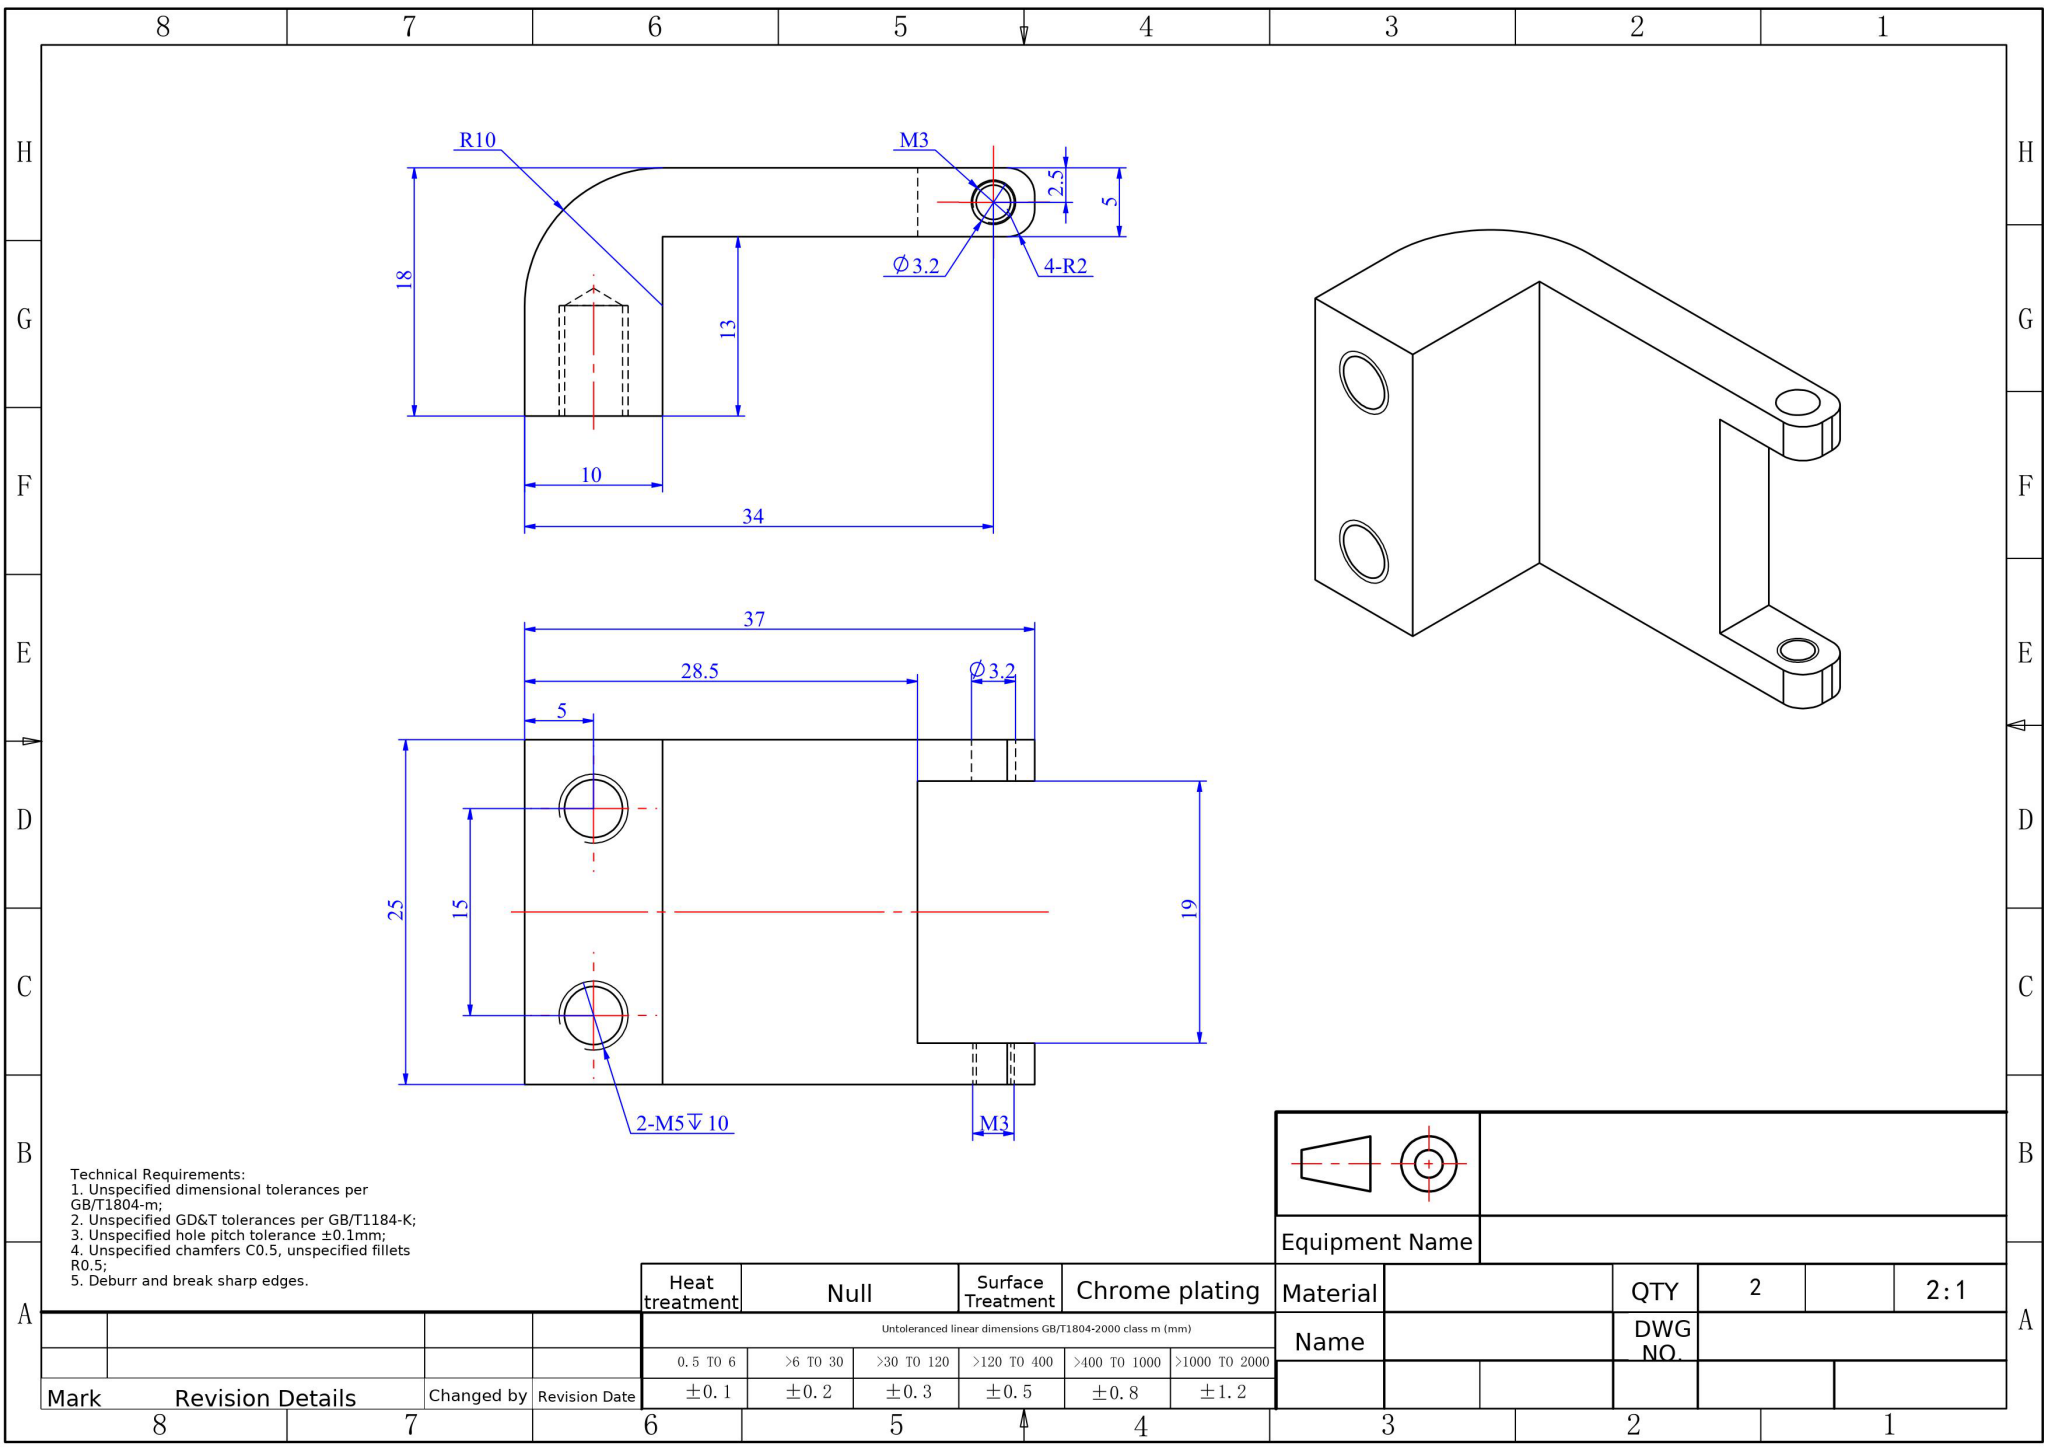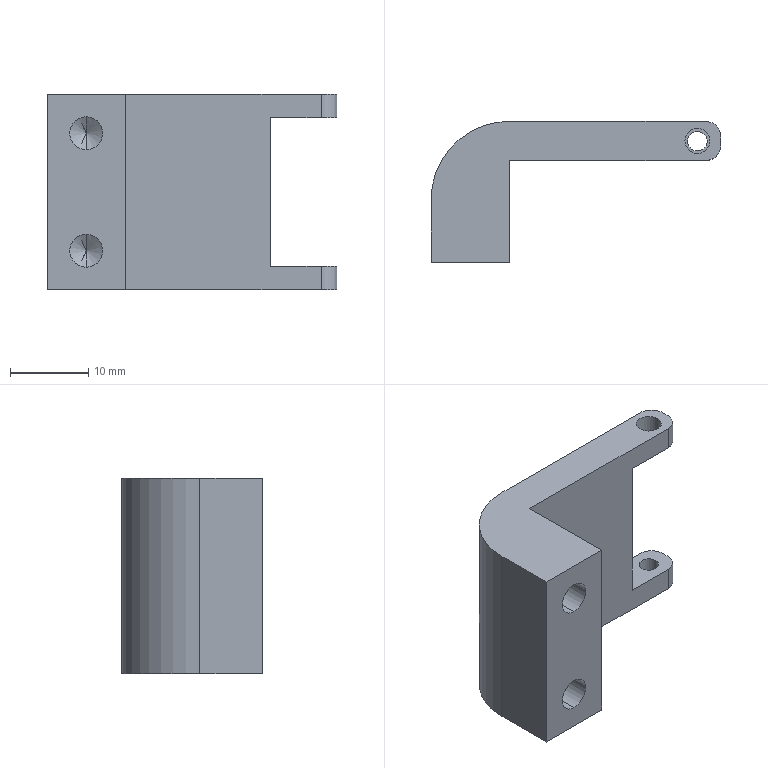Part | NX | mm | 1 solid | 29 faces | box 37 x 18 x 25 mm | volume 6249 mm3 | cylinder 13 | plane 12 | cone 4 | commonest cylinder face diameters 4.2 x4 4 x4 2.5 x2 3.2 x2 20 x1
STEP:
#1=COLOUR_RGB('',0.7922,0.8196,0.9333);
#2=FILL_AREA_STYLE_COLOUR('',#1);
#3=FILL_AREA_STYLE('',(#2));
#4=SURFACE_STYLE_FILL_AREA(#3);
#5=SURFACE_SIDE_STYLE('',(#4));
#6=SURFACE_STYLE_USAGE(.BOTH.,#5);
#7=PRESENTATION_STYLE_ASSIGNMENT((#6));
#8=CARTESIAN_POINT('',(32.75,15.498,-12.5));
#9=VERTEX_POINT('',#8);
#10=CARTESIAN_POINT('',(35.25,15.498,-12.5));
#11=VERTEX_POINT('',#10);
#12=CARTESIAN_POINT('',(34.,15.498,-12.5));
#13=DIRECTION('',(0.,0.,1.));
#14=DIRECTION('',(1.,0.,0.));
#15=AXIS2_PLACEMENT_3D('',#12,#13,#14);
#16=CIRCLE('',#15,1.25);
#17=EDGE_CURVE('',#9,#11,#16,.T.);
#18=ORIENTED_EDGE('',*,*,#17,.F.);
#19=CARTESIAN_POINT('',(32.75,15.498,-9.5));
#20=VERTEX_POINT('',#19);
#21=CARTESIAN_POINT('',(32.75,15.498,-9.5));
#22=DIRECTION('',(0.,0.,1.));
#23=VECTOR('',#22,1000.);
#24=LINE('',#21,#23);
#25=EDGE_CURVE('',#9,#20,#24,.T.);
#26=ORIENTED_EDGE('',*,*,#25,.T.);
#27=CARTESIAN_POINT('',(35.25,15.498,-9.5));
#28=VERTEX_POINT('',#27);
#29=CARTESIAN_POINT('',(34.,15.498,-9.5));
#30=DIRECTION('',(0.,0.,1.));
#31=DIRECTION('',(1.,0.,0.));
#32=AXIS2_PLACEMENT_3D('',#29,#30,#31);
#33=CIRCLE('',#32,1.25);
#34=EDGE_CURVE('',#20,#28,#33,.T.);
#35=ORIENTED_EDGE('',*,*,#34,.T.);
#36=CARTESIAN_POINT('',(35.25,15.498,-9.5));
#37=DIRECTION('',(0.,0.,1.));
#38=VECTOR('',#37,1000.);
#39=LINE('',#36,#38);
#40=EDGE_CURVE('',#11,#28,#39,.T.);
#41=ORIENTED_EDGE('',*,*,#40,.F.);
#42=EDGE_LOOP('',(#18,#26,#35,#41));
#43=FACE_OUTER_BOUND('',#42,.T.);
#44=CARTESIAN_POINT('',(34.,15.498,-9.5));
#45=DIRECTION('',(0.,0.,1.));
#46=DIRECTION('',(1.,0.,0.));
#47=AXIS2_PLACEMENT_3D('',#44,#45,#46);
#48=CYLINDRICAL_SURFACE('',#47,1.25);
#49=ADVANCED_FACE('',(#43),#48,.F.);
#50=CARTESIAN_POINT('',(5.,8.,9.6));
#51=VERTEX_POINT('',#50);
#52=CARTESIAN_POINT('',(5.,8.,5.4));
#53=VERTEX_POINT('',#52);
#54=CARTESIAN_POINT('',(5.,8.,7.5));
#55=DIRECTION('',(0.,-1.,0.));
#56=DIRECTION('',(0.,0.,-1.));
#57=AXIS2_PLACEMENT_3D('',#54,#55,#56);
#58=CIRCLE('',#57,2.1);
#59=EDGE_CURVE('',#51,#53,#58,.T.);
#60=ORIENTED_EDGE('',*,*,#59,.F.);
#61=CARTESIAN_POINT('',(5.,0.,9.6));
#62=VERTEX_POINT('',#61);
#63=CARTESIAN_POINT('',(5.,0.,9.6));
#64=DIRECTION('',(0.,-1.,0.));
#65=VECTOR('',#64,1000.);
#66=LINE('',#63,#65);
#67=EDGE_CURVE('',#51,#62,#66,.T.);
#68=ORIENTED_EDGE('',*,*,#67,.T.);
#69=CARTESIAN_POINT('',(5.,0.,5.4));
#70=VERTEX_POINT('',#69);
#71=CARTESIAN_POINT('',(5.,0.,7.5));
#72=DIRECTION('',(0.,-1.,0.));
#73=DIRECTION('',(0.,0.,-1.));
#74=AXIS2_PLACEMENT_3D('',#71,#72,#73);
#75=CIRCLE('',#74,2.1);
#76=EDGE_CURVE('',#62,#70,#75,.T.);
#77=ORIENTED_EDGE('',*,*,#76,.T.);
#78=CARTESIAN_POINT('',(5.,0.,5.4));
#79=DIRECTION('',(0.,-1.,0.));
#80=VECTOR('',#79,1000.);
#81=LINE('',#78,#80);
#82=EDGE_CURVE('',#53,#70,#81,.T.);
#83=ORIENTED_EDGE('',*,*,#82,.F.);
#84=EDGE_LOOP('',(#60,#68,#77,#83));
#85=FACE_OUTER_BOUND('',#84,.T.);
#86=CARTESIAN_POINT('',(5.,0.,7.5));
#87=DIRECTION('',(0.,-1.,0.));
#88=DIRECTION('',(0.,0.,-1.));
#89=AXIS2_PLACEMENT_3D('',#86,#87,#88);
#90=CYLINDRICAL_SURFACE('',#89,2.1);
#91=ADVANCED_FACE('',(#85),#90,.F.);
#92=CARTESIAN_POINT('',(5.,9.262,7.5));
#93=VERTEX_POINT('',#92);
#94=CARTESIAN_POINT('',(5.,8.,5.4));
#95=DIRECTION('',(0.,-0.515,-0.8572));
#96=VECTOR('',#95,1000.);
#97=LINE('',#94,#96);
#98=EDGE_CURVE('',#93,#53,#97,.T.);
#99=ORIENTED_EDGE('',*,*,#98,.F.);
#100=CARTESIAN_POINT('',(5.,8.,9.6));
#101=DIRECTION('',(0.,-0.515,0.8572));
#102=VECTOR('',#101,1000.);
#103=LINE('',#100,#102);
#104=EDGE_CURVE('',#93,#51,#103,.T.);
#105=ORIENTED_EDGE('',*,*,#104,.T.);
#106=ORIENTED_EDGE('',*,*,#59,.T.);
#107=EDGE_LOOP('',(#99,#105,#106));
#108=FACE_OUTER_BOUND('',#107,.T.);
#109=CARTESIAN_POINT('',(5.,8.,7.5));
#110=DIRECTION('',(0.,-1.,0.));
#111=DIRECTION('',(0.,0.,-1.));
#112=AXIS2_PLACEMENT_3D('',#109,#110,#111);
#113=CONICAL_SURFACE('',#112,2.1,1.03);
#114=ADVANCED_FACE('',(#108),#113,.F.);
#115=CARTESIAN_POINT('',(5.,8.,-5.4));
#116=VERTEX_POINT('',#115);
#117=CARTESIAN_POINT('',(5.,8.,-9.6));
#118=VERTEX_POINT('',#117);
#119=CARTESIAN_POINT('',(5.,8.,-7.5));
#120=DIRECTION('',(0.,-1.,0.));
#121=DIRECTION('',(0.,0.,-1.));
#122=AXIS2_PLACEMENT_3D('',#119,#120,#121);
#123=CIRCLE('',#122,2.1);
#124=EDGE_CURVE('',#116,#118,#123,.T.);
#125=ORIENTED_EDGE('',*,*,#124,.F.);
#126=CARTESIAN_POINT('',(5.,0.,-5.4));
#127=VERTEX_POINT('',#126);
#128=CARTESIAN_POINT('',(5.,0.,-5.4));
#129=DIRECTION('',(0.,-1.,0.));
#130=VECTOR('',#129,1000.);
#131=LINE('',#128,#130);
#132=EDGE_CURVE('',#116,#127,#131,.T.);
#133=ORIENTED_EDGE('',*,*,#132,.T.);
#134=CARTESIAN_POINT('',(5.,0.,-9.6));
#135=VERTEX_POINT('',#134);
#136=CARTESIAN_POINT('',(5.,0.,-7.5));
#137=DIRECTION('',(0.,-1.,0.));
#138=DIRECTION('',(0.,0.,-1.));
#139=AXIS2_PLACEMENT_3D('',#136,#137,#138);
#140=CIRCLE('',#139,2.1);
#141=EDGE_CURVE('',#127,#135,#140,.T.);
#142=ORIENTED_EDGE('',*,*,#141,.T.);
#143=CARTESIAN_POINT('',(5.,0.,-9.6));
#144=DIRECTION('',(0.,-1.,0.));
#145=VECTOR('',#144,1000.);
#146=LINE('',#143,#145);
#147=EDGE_CURVE('',#118,#135,#146,.T.);
#148=ORIENTED_EDGE('',*,*,#147,.F.);
#149=EDGE_LOOP('',(#125,#133,#142,#148));
#150=FACE_OUTER_BOUND('',#149,.T.);
#151=CARTESIAN_POINT('',(5.,0.,-7.5));
#152=DIRECTION('',(0.,-1.,0.));
#153=DIRECTION('',(0.,0.,-1.));
#154=AXIS2_PLACEMENT_3D('',#151,#152,#153);
#155=CYLINDRICAL_SURFACE('',#154,2.1);
#156=ADVANCED_FACE('',(#150),#155,.F.);
#157=CARTESIAN_POINT('',(5.,9.262,-7.5));
#158=VERTEX_POINT('',#157);
#159=CARTESIAN_POINT('',(5.,8.,-9.6));
#160=DIRECTION('',(0.,-0.515,-0.8572));
#161=VECTOR('',#160,1000.);
#162=LINE('',#159,#161);
#163=EDGE_CURVE('',#158,#118,#162,.T.);
#164=ORIENTED_EDGE('',*,*,#163,.F.);
#165=CARTESIAN_POINT('',(5.,8.,-5.4));
#166=DIRECTION('',(0.,-0.515,0.8572));
#167=VECTOR('',#166,1000.);
#168=LINE('',#165,#167);
#169=EDGE_CURVE('',#158,#116,#168,.T.);
#170=ORIENTED_EDGE('',*,*,#169,.T.);
#171=ORIENTED_EDGE('',*,*,#124,.T.);
#172=EDGE_LOOP('',(#164,#170,#171));
#173=FACE_OUTER_BOUND('',#172,.T.);
#174=CARTESIAN_POINT('',(5.,8.,-7.5));
#175=DIRECTION('',(0.,-1.,0.));
#176=DIRECTION('',(0.,0.,-1.));
#177=AXIS2_PLACEMENT_3D('',#174,#175,#176);
#178=CONICAL_SURFACE('',#177,2.1,1.03);
#179=ADVANCED_FACE('',(#173),#178,.F.);
#180=CARTESIAN_POINT('',(32.4,15.498,9.5));
#181=VERTEX_POINT('',#180);
#182=CARTESIAN_POINT('',(35.6,15.498,9.5));
#183=VERTEX_POINT('',#182);
#184=CARTESIAN_POINT('',(34.,15.498,9.5));
#185=DIRECTION('',(0.,0.,1.));
#186=DIRECTION('',(1.,0.,0.));
#187=AXIS2_PLACEMENT_3D('',#184,#185,#186);
#188=CIRCLE('',#187,1.6);
#189=EDGE_CURVE('',#181,#183,#188,.T.);
#190=ORIENTED_EDGE('',*,*,#189,.F.);
#191=CARTESIAN_POINT('',(32.4,15.498,12.5));
#192=VERTEX_POINT('',#191);
#193=CARTESIAN_POINT('',(32.4,15.498,12.5));
#194=DIRECTION('',(0.,0.,1.));
#195=VECTOR('',#194,1000.);
#196=LINE('',#193,#195);
#197=EDGE_CURVE('',#181,#192,#196,.T.);
#198=ORIENTED_EDGE('',*,*,#197,.T.);
#199=CARTESIAN_POINT('',(35.6,15.498,12.5));
#200=VERTEX_POINT('',#199);
#201=CARTESIAN_POINT('',(34.,15.498,12.5));
#202=DIRECTION('',(0.,0.,1.));
#203=DIRECTION('',(1.,0.,0.));
#204=AXIS2_PLACEMENT_3D('',#201,#202,#203);
#205=CIRCLE('',#204,1.6);
#206=EDGE_CURVE('',#192,#200,#205,.T.);
#207=ORIENTED_EDGE('',*,*,#206,.T.);
#208=CARTESIAN_POINT('',(35.6,15.498,12.5));
#209=DIRECTION('',(0.,0.,1.));
#210=VECTOR('',#209,1000.);
#211=LINE('',#208,#210);
#212=EDGE_CURVE('',#183,#200,#211,.T.);
#213=ORIENTED_EDGE('',*,*,#212,.F.);
#214=EDGE_LOOP('',(#190,#198,#207,#213));
#215=FACE_OUTER_BOUND('',#214,.T.);
#216=CARTESIAN_POINT('',(34.,15.498,12.5));
#217=DIRECTION('',(0.,0.,1.));
#218=DIRECTION('',(1.,0.,0.));
#219=AXIS2_PLACEMENT_3D('',#216,#217,#218);
#220=CYLINDRICAL_SURFACE('',#219,1.6);
#221=ADVANCED_FACE('',(#215),#220,.F.);
#222=CARTESIAN_POINT('',(10.,13.,12.5));
#223=VERTEX_POINT('',#222);
#224=CARTESIAN_POINT('',(35.,13.,12.5));
#225=VERTEX_POINT('',#224);
#226=CARTESIAN_POINT('',(10.,13.,12.5));
#227=DIRECTION('',(1.,-0.,0.));
#228=VECTOR('',#227,1000.);
#229=LINE('',#226,#228);
#230=EDGE_CURVE('',#223,#225,#229,.T.);
#231=ORIENTED_EDGE('',*,*,#230,.T.);
#232=CARTESIAN_POINT('',(37.,15.,12.5));
#233=VERTEX_POINT('',#232);
#234=CARTESIAN_POINT('',(35.,15.,12.5));
#235=DIRECTION('',(0.,0.,1.));
#236=DIRECTION('',(-1.,0.,0.));
#237=AXIS2_PLACEMENT_3D('',#234,#235,#236);
#238=CIRCLE('',#237,2.);
#239=EDGE_CURVE('',#225,#233,#238,.T.);
#240=ORIENTED_EDGE('',*,*,#239,.T.);
#241=CARTESIAN_POINT('',(37.,16.,12.5));
#242=VERTEX_POINT('',#241);
#243=CARTESIAN_POINT('',(37.,13.,12.5));
#244=DIRECTION('',(0.,1.,0.));
#245=VECTOR('',#244,1000.);
#246=LINE('',#243,#245);
#247=EDGE_CURVE('',#233,#242,#246,.T.);
#248=ORIENTED_EDGE('',*,*,#247,.T.);
#249=CARTESIAN_POINT('',(35.,18.,12.5));
#250=VERTEX_POINT('',#249);
#251=CARTESIAN_POINT('',(35.,16.,12.5));
#252=DIRECTION('',(0.,0.,1.));
#253=DIRECTION('',(-1.,0.,0.));
#254=AXIS2_PLACEMENT_3D('',#251,#252,#253);
#255=CIRCLE('',#254,2.);
#256=EDGE_CURVE('',#242,#250,#255,.T.);
#257=ORIENTED_EDGE('',*,*,#256,.T.);
#258=CARTESIAN_POINT('',(10.,18.,12.5));
#259=VERTEX_POINT('',#258);
#260=CARTESIAN_POINT('',(37.,18.,12.5));
#261=DIRECTION('',(-1.,-0.,0.));
#262=VECTOR('',#261,1000.);
#263=LINE('',#260,#262);
#264=EDGE_CURVE('',#250,#259,#263,.T.);
#265=ORIENTED_EDGE('',*,*,#264,.T.);
#266=CARTESIAN_POINT('',(0.,8.,12.5));
#267=VERTEX_POINT('',#266);
#268=CARTESIAN_POINT('',(10.,8.,12.5));
#269=DIRECTION('',(0.,0.,1.));
#270=DIRECTION('',(-1.,0.,0.));
#271=AXIS2_PLACEMENT_3D('',#268,#269,#270);
#272=CIRCLE('',#271,10.);
#273=EDGE_CURVE('',#259,#267,#272,.T.);
#274=ORIENTED_EDGE('',*,*,#273,.T.);
#275=CARTESIAN_POINT('',(0.,0.,12.5));
#276=VERTEX_POINT('',#275);
#277=CARTESIAN_POINT('',(-0.,8.,12.5));
#278=DIRECTION('',(0.,-1.,0.));
#279=VECTOR('',#278,1000.);
#280=LINE('',#277,#279);
#281=EDGE_CURVE('',#267,#276,#280,.T.);
#282=ORIENTED_EDGE('',*,*,#281,.T.);
#283=CARTESIAN_POINT('',(10.,0.,12.5));
#284=VERTEX_POINT('',#283);
#285=CARTESIAN_POINT('',(0.,0.,12.5));
#286=DIRECTION('',(1.,0.,0.));
#287=VECTOR('',#286,1000.);
#288=LINE('',#285,#287);
#289=EDGE_CURVE('',#276,#284,#288,.T.);
#290=ORIENTED_EDGE('',*,*,#289,.T.);
#291=CARTESIAN_POINT('',(10.,0.,12.5));
#292=DIRECTION('',(-0.,1.,0.));
#293=VECTOR('',#292,1000.);
#294=LINE('',#291,#293);
#295=EDGE_CURVE('',#284,#223,#294,.T.);
#296=ORIENTED_EDGE('',*,*,#295,.T.);
#297=EDGE_LOOP('',(#231,#240,#248,#257,#265,#274,#282,#290,#296));
#298=FACE_OUTER_BOUND('',#297,.T.);
#299=CARTESIAN_POINT('',(34.,15.498,12.5));
#300=DIRECTION('',(0.,0.,1.));
#301=DIRECTION('',(1.,0.,0.));
#302=AXIS2_PLACEMENT_3D('',#299,#300,#301);
#303=CIRCLE('',#302,1.6);
#304=EDGE_CURVE('',#200,#192,#303,.T.);
#305=ORIENTED_EDGE('',*,*,#304,.F.);
#306=ORIENTED_EDGE('',*,*,#206,.F.);
#307=EDGE_LOOP('',(#305,#306));
#308=FACE_BOUND('',#307,.T.);
#309=CARTESIAN_POINT('',(10.,8.,12.5));
#310=DIRECTION('',(0.,0.,-1.));
#311=DIRECTION('',(-1.,0.,0.));
#312=AXIS2_PLACEMENT_3D('',#309,#310,#311);
#313=PLANE('',#312);
#314=ADVANCED_FACE('',(#298,#308),#313,.F.);
#315=ORIENTED_EDGE('',*,*,#247,.F.);
#316=CARTESIAN_POINT('',(37.,15.,9.5));
#317=VERTEX_POINT('',#316);
#318=CARTESIAN_POINT('',(37.,15.,12.5));
#319=DIRECTION('',(0.,0.,-1.));
#320=VECTOR('',#319,1000.);
#321=LINE('',#318,#320);
#322=EDGE_CURVE('',#233,#317,#321,.T.);
#323=ORIENTED_EDGE('',*,*,#322,.T.);
#324=CARTESIAN_POINT('',(37.,16.,9.5));
#325=VERTEX_POINT('',#324);
#326=CARTESIAN_POINT('',(37.,-7.,9.5));
#327=DIRECTION('',(-0.,1.,0.));
#328=VECTOR('',#327,1000.);
#329=LINE('',#326,#328);
#330=EDGE_CURVE('',#317,#325,#329,.T.);
#331=ORIENTED_EDGE('',*,*,#330,.T.);
#332=CARTESIAN_POINT('',(37.,16.,12.5));
#333=DIRECTION('',(0.,0.,1.));
#334=VECTOR('',#333,1000.);
#335=LINE('',#332,#334);
#336=EDGE_CURVE('',#325,#242,#335,.T.);
#337=ORIENTED_EDGE('',*,*,#336,.T.);
#338=EDGE_LOOP('',(#315,#323,#331,#337));
#339=FACE_OUTER_BOUND('',#338,.T.);
#340=CARTESIAN_POINT('',(37.,13.,12.5));
#341=DIRECTION('',(-1.,0.,0.));
#342=DIRECTION('',(0.,0.,1.));
#343=AXIS2_PLACEMENT_3D('',#340,#341,#342);
#344=PLANE('',#343);
#345=ADVANCED_FACE('',(#339),#344,.F.);
#346=CARTESIAN_POINT('',(0.,8.,-12.5));
#347=VERTEX_POINT('',#346);
#348=CARTESIAN_POINT('',(0.,0.,-12.5));
#349=VERTEX_POINT('',#348);
#350=CARTESIAN_POINT('',(-0.,8.,-12.5));
#351=DIRECTION('',(0.,-1.,0.));
#352=VECTOR('',#351,1000.);
#353=LINE('',#350,#352);
#354=EDGE_CURVE('',#347,#349,#353,.T.);
#355=ORIENTED_EDGE('',*,*,#354,.T.);
#356=CARTESIAN_POINT('',(0.,0.,12.5));
#357=DIRECTION('',(0.,0.,-1.));
#358=VECTOR('',#357,1000.);
#359=LINE('',#356,#358);
#360=EDGE_CURVE('',#276,#349,#359,.T.);
#361=ORIENTED_EDGE('',*,*,#360,.F.);
#362=ORIENTED_EDGE('',*,*,#281,.F.);
#363=CARTESIAN_POINT('',(0.,8.,12.5));
#364=DIRECTION('',(0.,0.,-1.));
#365=VECTOR('',#364,1000.);
#366=LINE('',#363,#365);
#367=EDGE_CURVE('',#267,#347,#366,.T.);
#368=ORIENTED_EDGE('',*,*,#367,.T.);
#369=EDGE_LOOP('',(#355,#361,#362,#368));
#370=FACE_OUTER_BOUND('',#369,.T.);
#371=CARTESIAN_POINT('',(-0.,8.,12.5));
#372=DIRECTION('',(1.,0.,0.));
#373=DIRECTION('',(-0.,1.,0.));
#374=AXIS2_PLACEMENT_3D('',#371,#372,#373);
#375=PLANE('',#374);
#376=ADVANCED_FACE('',(#370),#375,.F.);
#377=CARTESIAN_POINT('',(5.,0.,7.5));
#378=DIRECTION('',(0.,-1.,0.));
#379=DIRECTION('',(0.,0.,-1.));
#380=AXIS2_PLACEMENT_3D('',#377,#378,#379);
#381=CIRCLE('',#380,2.1);
#382=EDGE_CURVE('',#70,#62,#381,.T.);
#383=ORIENTED_EDGE('',*,*,#382,.F.);
#384=ORIENTED_EDGE('',*,*,#76,.F.);
#385=EDGE_LOOP('',(#383,#384));
#386=FACE_BOUND('',#385,.T.);
#387=CARTESIAN_POINT('',(5.,0.,-7.5));
#388=DIRECTION('',(0.,-1.,0.));
#389=DIRECTION('',(0.,0.,-1.));
#390=AXIS2_PLACEMENT_3D('',#387,#388,#389);
#391=CIRCLE('',#390,2.1);
#392=EDGE_CURVE('',#135,#127,#391,.T.);
#393=ORIENTED_EDGE('',*,*,#392,.F.);
#394=ORIENTED_EDGE('',*,*,#141,.F.);
#395=EDGE_LOOP('',(#393,#394));
#396=FACE_BOUND('',#395,.T.);
#397=CARTESIAN_POINT('',(10.,0.,-12.5));
#398=VERTEX_POINT('',#397);
#399=CARTESIAN_POINT('',(0.,0.,-12.5));
#400=DIRECTION('',(1.,0.,0.));
#401=VECTOR('',#400,1000.);
#402=LINE('',#399,#401);
#403=EDGE_CURVE('',#349,#398,#402,.T.);
#404=ORIENTED_EDGE('',*,*,#403,.T.);
#405=CARTESIAN_POINT('',(10.,0.,12.5));
#406=DIRECTION('',(0.,0.,-1.));
#407=VECTOR('',#406,1000.);
#408=LINE('',#405,#407);
#409=EDGE_CURVE('',#284,#398,#408,.T.);
#410=ORIENTED_EDGE('',*,*,#409,.F.);
#411=ORIENTED_EDGE('',*,*,#289,.F.);
#412=ORIENTED_EDGE('',*,*,#360,.T.);
#413=EDGE_LOOP('',(#404,#410,#411,#412));
#414=FACE_OUTER_BOUND('',#413,.T.);
#415=CARTESIAN_POINT('',(0.,0.,12.5));
#416=DIRECTION('',(0.,1.,0.));
#417=DIRECTION('',(0.,0.,1.));
#418=AXIS2_PLACEMENT_3D('',#415,#416,#417);
#419=PLANE('',#418);
#420=ADVANCED_FACE('',(#386,#396,#414),#419,.F.);
#421=CARTESIAN_POINT('',(10.,13.,-12.5));
#422=VERTEX_POINT('',#421);
#423=CARTESIAN_POINT('',(10.,0.,-12.5));
#424=DIRECTION('',(-0.,1.,0.));
#425=VECTOR('',#424,1000.);
#426=LINE('',#423,#425);
#427=EDGE_CURVE('',#398,#422,#426,.T.);
#428=ORIENTED_EDGE('',*,*,#427,.T.);
#429=CARTESIAN_POINT('',(10.,13.,12.5));
#430=DIRECTION('',(0.,0.,-1.));
#431=VECTOR('',#430,1000.);
#432=LINE('',#429,#431);
#433=EDGE_CURVE('',#223,#422,#432,.T.);
#434=ORIENTED_EDGE('',*,*,#433,.F.);
#435=ORIENTED_EDGE('',*,*,#295,.F.);
#436=ORIENTED_EDGE('',*,*,#409,.T.);
#437=EDGE_LOOP('',(#428,#434,#435,#436));
#438=FACE_OUTER_BOUND('',#437,.T.);
#439=CARTESIAN_POINT('',(10.,0.,12.5));
#440=DIRECTION('',(-1.,-0.,0.));
#441=DIRECTION('',(0.,-1.,0.));
#442=AXIS2_PLACEMENT_3D('',#439,#440,#441);
#443=PLANE('',#442);
#444=ADVANCED_FACE('',(#438),#443,.F.);
#445=CARTESIAN_POINT('',(35.,13.,-12.5));
#446=VERTEX_POINT('',#445);
#447=CARTESIAN_POINT('',(10.,13.,-12.5));
#448=DIRECTION('',(1.,-0.,0.));
#449=VECTOR('',#448,1000.);
#450=LINE('',#447,#449);
#451=EDGE_CURVE('',#422,#446,#450,.T.);
#452=ORIENTED_EDGE('',*,*,#451,.T.);
#453=CARTESIAN_POINT('',(35.,13.,-9.5));
#454=VERTEX_POINT('',#453);
#455=CARTESIAN_POINT('',(35.,13.,12.5));
#456=DIRECTION('',(0.,0.,1.));
#457=VECTOR('',#456,1000.);
#458=LINE('',#455,#457);
#459=EDGE_CURVE('',#446,#454,#458,.T.);
#460=ORIENTED_EDGE('',*,*,#459,.T.);
#461=CARTESIAN_POINT('',(28.5,13.,-9.5));
#462=VERTEX_POINT('',#461);
#463=CARTESIAN_POINT('',(10.,13.,-9.5));
#464=DIRECTION('',(-1.,0.,0.));
#465=VECTOR('',#464,1000.);
#466=LINE('',#463,#465);
#467=EDGE_CURVE('',#454,#462,#466,.T.);
#468=ORIENTED_EDGE('',*,*,#467,.T.);
#469=CARTESIAN_POINT('',(28.5,13.,9.5));
#470=VERTEX_POINT('',#469);
#471=CARTESIAN_POINT('',(28.5,13.,12.5));
#472=DIRECTION('',(0.,0.,1.));
#473=VECTOR('',#472,1000.);
#474=LINE('',#471,#473);
#475=EDGE_CURVE('',#462,#470,#474,.T.);
#476=ORIENTED_EDGE('',*,*,#475,.T.);
#477=CARTESIAN_POINT('',(35.,13.,9.5));
#478=VERTEX_POINT('',#477);
#479=CARTESIAN_POINT('',(10.,13.,9.5));
#480=DIRECTION('',(1.,-0.,0.));
#481=VECTOR('',#480,1000.);
#482=LINE('',#479,#481);
#483=EDGE_CURVE('',#470,#478,#482,.T.);
#484=ORIENTED_EDGE('',*,*,#483,.T.);
#485=CARTESIAN_POINT('',(35.,13.,12.5));
#486=DIRECTION('',(0.,0.,1.));
#487=VECTOR('',#486,1000.);
#488=LINE('',#485,#487);
#489=EDGE_CURVE('',#478,#225,#488,.T.);
#490=ORIENTED_EDGE('',*,*,#489,.T.);
#491=ORIENTED_EDGE('',*,*,#230,.F.);
#492=ORIENTED_EDGE('',*,*,#433,.T.);
#493=EDGE_LOOP('',(#452,#460,#468,#476,#484,#490,#491,#492));
#494=FACE_OUTER_BOUND('',#493,.T.);
#495=CARTESIAN_POINT('',(10.,13.,12.5));
#496=DIRECTION('',(0.,1.,0.));
#497=DIRECTION('',(-1.,0.,0.));
#498=AXIS2_PLACEMENT_3D('',#495,#496,#497);
#499=PLANE('',#498);
#500=ADVANCED_FACE('',(#494),#499,.F.);
#501=CARTESIAN_POINT('',(37.,15.,-12.5));
#502=VERTEX_POINT('',#501);
#503=CARTESIAN_POINT('',(37.,16.,-12.5));
#504=VERTEX_POINT('',#503);
#505=CARTESIAN_POINT('',(37.,13.,-12.5));
#506=DIRECTION('',(0.,1.,0.));
#507=VECTOR('',#506,1000.);
#508=LINE('',#505,#507);
#509=EDGE_CURVE('',#502,#504,#508,.T.);
#510=ORIENTED_EDGE('',*,*,#509,.T.);
#511=CARTESIAN_POINT('',(37.,16.,-9.5));
#512=VERTEX_POINT('',#511);
#513=CARTESIAN_POINT('',(37.,16.,12.5));
#514=DIRECTION('',(0.,0.,1.));
#515=VECTOR('',#514,1000.);
#516=LINE('',#513,#515);
#517=EDGE_CURVE('',#504,#512,#516,.T.);
#518=ORIENTED_EDGE('',*,*,#517,.T.);
#519=CARTESIAN_POINT('',(37.,15.,-9.5));
#520=VERTEX_POINT('',#519);
#521=CARTESIAN_POINT('',(37.,-7.,-9.5));
#522=DIRECTION('',(-0.,1.,0.));
#523=VECTOR('',#522,1000.);
#524=LINE('',#521,#523);
#525=EDGE_CURVE('',#520,#512,#524,.T.);
#526=ORIENTED_EDGE('',*,*,#525,.F.);
#527=CARTESIAN_POINT('',(37.,15.,12.5));
#528=DIRECTION('',(0.,0.,-1.));
#529=VECTOR('',#528,1000.);
#530=LINE('',#527,#529);
#531=EDGE_CURVE('',#520,#502,#530,.T.);
#532=ORIENTED_EDGE('',*,*,#531,.T.);
#533=EDGE_LOOP('',(#510,#518,#526,#532));
#534=FACE_OUTER_BOUND('',#533,.T.);
#535=CARTESIAN_POINT('',(37.,13.,12.5));
#536=DIRECTION('',(-1.,0.,0.));
#537=DIRECTION('',(0.,0.,1.));
#538=AXIS2_PLACEMENT_3D('',#535,#536,#537);
#539=PLANE('',#538);
#540=ADVANCED_FACE('',(#534),#539,.F.);
#541=CARTESIAN_POINT('',(35.,18.,-9.5));
#542=VERTEX_POINT('',#541);
#543=CARTESIAN_POINT('',(28.5,18.,-9.5));
#544=VERTEX_POINT('',#543);
#545=CARTESIAN_POINT('',(37.,18.,-9.5));
#546=DIRECTION('',(-1.,0.,0.));
#547=VECTOR('',#546,1000.);
#548=LINE('',#545,#547);
#549=EDGE_CURVE('',#542,#544,#548,.T.);
#550=ORIENTED_EDGE('',*,*,#549,.F.);
#551=CARTESIAN_POINT('',(35.,18.,-12.5));
#552=VERTEX_POINT('',#551);
#553=CARTESIAN_POINT('',(35.,18.,12.5));
#554=DIRECTION('',(0.,0.,-1.));
#555=VECTOR('',#554,1000.);
#556=LINE('',#553,#555);
#557=EDGE_CURVE('',#542,#552,#556,.T.);
#558=ORIENTED_EDGE('',*,*,#557,.T.);
#559=CARTESIAN_POINT('',(10.,18.,-12.5));
#560=VERTEX_POINT('',#559);
#561=CARTESIAN_POINT('',(37.,18.,-12.5));
#562=DIRECTION('',(-1.,-0.,0.));
#563=VECTOR('',#562,1000.);
#564=LINE('',#561,#563);
#565=EDGE_CURVE('',#552,#560,#564,.T.);
#566=ORIENTED_EDGE('',*,*,#565,.T.);
#567=CARTESIAN_POINT('',(10.,18.,12.5));
#568=DIRECTION('',(0.,0.,-1.));
#569=VECTOR('',#568,1000.);
#570=LINE('',#567,#569);
#571=EDGE_CURVE('',#259,#560,#570,.T.);
#572=ORIENTED_EDGE('',*,*,#571,.F.);
#573=ORIENTED_EDGE('',*,*,#264,.F.);
#574=CARTESIAN_POINT('',(35.,18.,9.5));
#575=VERTEX_POINT('',#574);
#576=CARTESIAN_POINT('',(35.,18.,12.5));
#577=DIRECTION('',(0.,0.,-1.));
#578=VECTOR('',#577,1000.);
#579=LINE('',#576,#578);
#580=EDGE_CURVE('',#250,#575,#579,.T.);
#581=ORIENTED_EDGE('',*,*,#580,.T.);
#582=CARTESIAN_POINT('',(28.5,18.,9.5));
#583=VERTEX_POINT('',#582);
#584=CARTESIAN_POINT('',(37.,18.,9.5));
#585=DIRECTION('',(1.,0.,0.));
#586=VECTOR('',#585,1000.);
#587=LINE('',#584,#586);
#588=EDGE_CURVE('',#583,#575,#587,.T.);
#589=ORIENTED_EDGE('',*,*,#588,.F.);
#590=CARTESIAN_POINT('',(28.5,18.,-9.5));
#591=DIRECTION('',(0.,0.,1.));
#592=VECTOR('',#591,1000.);
#593=LINE('',#590,#592);
#594=EDGE_CURVE('',#544,#583,#593,.T.);
#595=ORIENTED_EDGE('',*,*,#594,.F.);
#596=EDGE_LOOP('',(#550,#558,#566,#572,#573,#581,#589,#595));
#597=FACE_OUTER_BOUND('',#596,.T.);
#598=CARTESIAN_POINT('',(37.,18.,12.5));
#599=DIRECTION('',(0.,-1.,0.));
#600=DIRECTION('',(1.,0.,0.));
#601=AXIS2_PLACEMENT_3D('',#598,#599,#600);
#602=PLANE('',#601);
#603=ADVANCED_FACE('',(#597),#602,.F.);
#604=CARTESIAN_POINT('',(10.,8.,-12.5));
#605=DIRECTION('',(0.,0.,1.));
#606=DIRECTION('',(-1.,0.,0.));
#607=AXIS2_PLACEMENT_3D('',#604,#605,#606);
#608=CIRCLE('',#607,10.);
#609=EDGE_CURVE('',#560,#347,#608,.T.);
#610=ORIENTED_EDGE('',*,*,#609,.T.);
#611=ORIENTED_EDGE('',*,*,#367,.F.);
#612=ORIENTED_EDGE('',*,*,#273,.F.);
#613=ORIENTED_EDGE('',*,*,#571,.T.);
#614=EDGE_LOOP('',(#610,#611,#612,#613));
#615=FACE_OUTER_BOUND('',#614,.T.);
#616=CARTESIAN_POINT('',(10.,8.,12.5));
#617=DIRECTION('',(0.,0.,-1.));
#618=DIRECTION('',(-1.,0.,0.));
#619=AXIS2_PLACEMENT_3D('',#616,#617,#618);
#620=CYLINDRICAL_SURFACE('',#619,10.);
#621=ADVANCED_FACE('',(#615),#620,.T.);
#622=CARTESIAN_POINT('',(34.,15.498,-12.5));
#623=DIRECTION('',(0.,0.,1.));
#624=DIRECTION('',(1.,0.,0.));
#625=AXIS2_PLACEMENT_3D('',#622,#623,#624);
#626=CIRCLE('',#625,1.25);
#627=EDGE_CURVE('',#11,#9,#626,.T.);
#628=ORIENTED_EDGE('',*,*,#627,.T.);
#629=ORIENTED_EDGE('',*,*,#17,.T.);
#630=EDGE_LOOP('',(#628,#629));
#631=FACE_BOUND('',#630,.T.);
#632=ORIENTED_EDGE('',*,*,#565,.F.);
#633=CARTESIAN_POINT('',(35.,16.,-12.5));
#634=DIRECTION('',(0.,0.,-1.));
#635=DIRECTION('',(-1.,0.,0.));
#636=AXIS2_PLACEMENT_3D('',#633,#634,#635);
#637=CIRCLE('',#636,2.);
#638=EDGE_CURVE('',#552,#504,#637,.T.);
#639=ORIENTED_EDGE('',*,*,#638,.T.);
#640=ORIENTED_EDGE('',*,*,#509,.F.);
#641=CARTESIAN_POINT('',(35.,15.,-12.5));
#642=DIRECTION('',(0.,0.,-1.));
#643=DIRECTION('',(-1.,0.,0.));
#644=AXIS2_PLACEMENT_3D('',#641,#642,#643);
#645=CIRCLE('',#644,2.);
#646=EDGE_CURVE('',#502,#446,#645,.T.);
#647=ORIENTED_EDGE('',*,*,#646,.T.);
#648=ORIENTED_EDGE('',*,*,#451,.F.);
#649=ORIENTED_EDGE('',*,*,#427,.F.);
#650=ORIENTED_EDGE('',*,*,#403,.F.);
#651=ORIENTED_EDGE('',*,*,#354,.F.);
#652=ORIENTED_EDGE('',*,*,#609,.F.);
#653=EDGE_LOOP('',(#632,#639,#640,#647,#648,#649,#650,#651,#652));
#654=FACE_OUTER_BOUND('',#653,.T.);
#655=CARTESIAN_POINT('',(10.,8.,-12.5));
#656=DIRECTION('',(0.,0.,-1.));
#657=DIRECTION('',(-1.,0.,0.));
#658=AXIS2_PLACEMENT_3D('',#655,#656,#657);
#659=PLANE('',#658);
#660=ADVANCED_FACE('',(#631,#654),#659,.T.);
#661=CARTESIAN_POINT('',(34.,15.498,9.5));
#662=DIRECTION('',(0.,0.,1.));
#663=DIRECTION('',(1.,0.,0.));
#664=AXIS2_PLACEMENT_3D('',#661,#662,#663);
#665=CIRCLE('',#664,1.6);
#666=EDGE_CURVE('',#183,#181,#665,.T.);
#667=ORIENTED_EDGE('',*,*,#666,.T.);
#668=ORIENTED_EDGE('',*,*,#189,.T.);
#669=EDGE_LOOP('',(#667,#668));
#670=FACE_BOUND('',#669,.T.);
#671=ORIENTED_EDGE('',*,*,#330,.F.);
#672=CARTESIAN_POINT('',(35.,15.,9.5));
#673=DIRECTION('',(0.,0.,-1.));
#674=DIRECTION('',(1.,0.,0.));
#675=AXIS2_PLACEMENT_3D('',#672,#673,#674);
#676=CIRCLE('',#675,2.);
#677=EDGE_CURVE('',#317,#478,#676,.T.);
#678=ORIENTED_EDGE('',*,*,#677,.T.);
#679=ORIENTED_EDGE('',*,*,#483,.F.);
#680=CARTESIAN_POINT('',(28.5,-7.,9.5));
#681=DIRECTION('',(-0.,1.,0.));
#682=VECTOR('',#681,1000.);
#683=LINE('',#680,#682);
#684=EDGE_CURVE('',#470,#583,#683,.T.);
#685=ORIENTED_EDGE('',*,*,#684,.T.);
#686=ORIENTED_EDGE('',*,*,#588,.T.);
#687=CARTESIAN_POINT('',(35.,16.,9.5));
#688=DIRECTION('',(0.,0.,-1.));
#689=DIRECTION('',(1.,0.,0.));
#690=AXIS2_PLACEMENT_3D('',#687,#688,#689);
#691=CIRCLE('',#690,2.);
#692=EDGE_CURVE('',#575,#325,#691,.T.);
#693=ORIENTED_EDGE('',*,*,#692,.T.);
#694=EDGE_LOOP('',(#671,#678,#679,#685,#686,#693));
#695=FACE_OUTER_BOUND('',#694,.T.);
#696=CARTESIAN_POINT('',(37.,-7.,9.5));
#697=DIRECTION('',(0.,0.,1.));
#698=DIRECTION('',(1.,0.,0.));
#699=AXIS2_PLACEMENT_3D('',#696,#697,#698);
#700=PLANE('',#699);
#701=ADVANCED_FACE('',(#670,#695),#700,.F.);
#702=CARTESIAN_POINT('',(28.5,-7.,-9.5));
#703=DIRECTION('',(-0.,1.,0.));
#704=VECTOR('',#703,1000.);
#705=LINE('',#702,#704);
#706=EDGE_CURVE('',#462,#544,#705,.T.);
#707=ORIENTED_EDGE('',*,*,#706,.T.);
#708=ORIENTED_EDGE('',*,*,#594,.T.);
#709=ORIENTED_EDGE('',*,*,#684,.F.);
#710=ORIENTED_EDGE('',*,*,#475,.F.);
#711=EDGE_LOOP('',(#707,#708,#709,#710));
#712=FACE_OUTER_BOUND('',#711,.T.);
#713=CARTESIAN_POINT('',(28.5,-7.,-9.5));
#714=DIRECTION('',(-1.,-0.,0.));
#715=DIRECTION('',(0.,-1.,0.));
#716=AXIS2_PLACEMENT_3D('',#713,#714,#715);
#717=PLANE('',#716);
#718=ADVANCED_FACE('',(#712),#717,.F.);
#719=CARTESIAN_POINT('',(34.,15.498,-9.5));
#720=DIRECTION('',(0.,0.,1.));
#721=DIRECTION('',(1.,0.,0.));
#722=AXIS2_PLACEMENT_3D('',#719,#720,#721);
#723=CIRCLE('',#722,1.25);
#724=EDGE_CURVE('',#28,#20,#723,.T.);
#725=ORIENTED_EDGE('',*,*,#724,.F.);
#726=ORIENTED_EDGE('',*,*,#34,.F.);
#727=EDGE_LOOP('',(#725,#726));
#728=FACE_BOUND('',#727,.T.);
#729=ORIENTED_EDGE('',*,*,#525,.T.);
#730=CARTESIAN_POINT('',(35.,16.,-9.5));
#731=DIRECTION('',(0.,0.,1.));
#732=DIRECTION('',(-1.,0.,0.));
#733=AXIS2_PLACEMENT_3D('',#730,#731,#732);
#734=CIRCLE('',#733,2.);
#735=EDGE_CURVE('',#512,#542,#734,.T.);
#736=ORIENTED_EDGE('',*,*,#735,.T.);
#737=ORIENTED_EDGE('',*,*,#549,.T.);
#738=ORIENTED_EDGE('',*,*,#706,.F.);
#739=ORIENTED_EDGE('',*,*,#467,.F.);
#740=CARTESIAN_POINT('',(35.,15.,-9.5));
#741=DIRECTION('',(0.,0.,1.));
#742=DIRECTION('',(-1.,0.,0.));
#743=AXIS2_PLACEMENT_3D('',#740,#741,#742);
#744=CIRCLE('',#743,2.);
#745=EDGE_CURVE('',#454,#520,#744,.T.);
#746=ORIENTED_EDGE('',*,*,#745,.T.);
#747=EDGE_LOOP('',(#729,#736,#737,#738,#739,#746));
#748=FACE_OUTER_BOUND('',#747,.T.);
#749=CARTESIAN_POINT('',(37.,-7.,-9.5));
#750=DIRECTION('',(0.,0.,-1.));
#751=DIRECTION('',(-1.,0.,0.));
#752=AXIS2_PLACEMENT_3D('',#749,#750,#751);
#753=PLANE('',#752);
#754=ADVANCED_FACE('',(#728,#748),#753,.F.);
#755=ORIENTED_EDGE('',*,*,#197,.F.);
#756=ORIENTED_EDGE('',*,*,#666,.F.);
#757=ORIENTED_EDGE('',*,*,#212,.T.);
#758=ORIENTED_EDGE('',*,*,#304,.T.);
#759=EDGE_LOOP('',(#755,#756,#757,#758));
#760=FACE_OUTER_BOUND('',#759,.T.);
#761=CARTESIAN_POINT('',(34.,15.498,12.5));
#762=DIRECTION('',(0.,0.,1.));
#763=DIRECTION('',(1.,0.,0.));
#764=AXIS2_PLACEMENT_3D('',#761,#762,#763);
#765=CYLINDRICAL_SURFACE('',#764,1.6);
#766=ADVANCED_FACE('',(#760),#765,.F.);
#767=ORIENTED_EDGE('',*,*,#169,.F.);
#768=ORIENTED_EDGE('',*,*,#163,.T.);
#769=CARTESIAN_POINT('',(5.,8.,-7.5));
#770=DIRECTION('',(0.,-1.,0.));
#771=DIRECTION('',(0.,0.,-1.));
#772=AXIS2_PLACEMENT_3D('',#769,#770,#771);
#773=CIRCLE('',#772,2.1);
#774=EDGE_CURVE('',#118,#116,#773,.T.);
#775=ORIENTED_EDGE('',*,*,#774,.T.);
#776=EDGE_LOOP('',(#767,#768,#775));
#777=FACE_OUTER_BOUND('',#776,.T.);
#778=CARTESIAN_POINT('',(5.,8.,-7.5));
#779=DIRECTION('',(0.,-1.,0.));
#780=DIRECTION('',(0.,0.,-1.));
#781=AXIS2_PLACEMENT_3D('',#778,#779,#780);
#782=CONICAL_SURFACE('',#781,2.1,1.03);
#783=ADVANCED_FACE('',(#777),#782,.F.);
#784=ORIENTED_EDGE('',*,*,#132,.F.);
#785=ORIENTED_EDGE('',*,*,#774,.F.);
#786=ORIENTED_EDGE('',*,*,#147,.T.);
#787=ORIENTED_EDGE('',*,*,#392,.T.);
#788=EDGE_LOOP('',(#784,#785,#786,#787));
#789=FACE_OUTER_BOUND('',#788,.T.);
#790=CARTESIAN_POINT('',(5.,0.,-7.5));
#791=DIRECTION('',(0.,-1.,0.));
#792=DIRECTION('',(0.,0.,-1.));
#793=AXIS2_PLACEMENT_3D('',#790,#791,#792);
#794=CYLINDRICAL_SURFACE('',#793,2.1);
#795=ADVANCED_FACE('',(#789),#794,.F.);
#796=ORIENTED_EDGE('',*,*,#104,.F.);
#797=ORIENTED_EDGE('',*,*,#98,.T.);
#798=CARTESIAN_POINT('',(5.,8.,7.5));
#799=DIRECTION('',(0.,-1.,0.));
#800=DIRECTION('',(0.,0.,-1.));
#801=AXIS2_PLACEMENT_3D('',#798,#799,#800);
#802=CIRCLE('',#801,2.1);
#803=EDGE_CURVE('',#53,#51,#802,.T.);
#804=ORIENTED_EDGE('',*,*,#803,.T.);
#805=EDGE_LOOP('',(#796,#797,#804));
#806=FACE_OUTER_BOUND('',#805,.T.);
#807=CARTESIAN_POINT('',(5.,8.,7.5));
#808=DIRECTION('',(0.,-1.,0.));
#809=DIRECTION('',(0.,0.,-1.));
#810=AXIS2_PLACEMENT_3D('',#807,#808,#809);
#811=CONICAL_SURFACE('',#810,2.1,1.03);
#812=ADVANCED_FACE('',(#806),#811,.F.);
#813=ORIENTED_EDGE('',*,*,#67,.F.);
#814=ORIENTED_EDGE('',*,*,#803,.F.);
#815=ORIENTED_EDGE('',*,*,#82,.T.);
#816=ORIENTED_EDGE('',*,*,#382,.T.);
#817=EDGE_LOOP('',(#813,#814,#815,#816));
#818=FACE_OUTER_BOUND('',#817,.T.);
#819=CARTESIAN_POINT('',(5.,0.,7.5));
#820=DIRECTION('',(0.,-1.,0.));
#821=DIRECTION('',(0.,0.,-1.));
#822=AXIS2_PLACEMENT_3D('',#819,#820,#821);
#823=CYLINDRICAL_SURFACE('',#822,2.1);
#824=ADVANCED_FACE('',(#818),#823,.F.);
#825=ORIENTED_EDGE('',*,*,#735,.F.);
#826=ORIENTED_EDGE('',*,*,#517,.F.);
#827=ORIENTED_EDGE('',*,*,#638,.F.);
#828=ORIENTED_EDGE('',*,*,#557,.F.);
#829=EDGE_LOOP('',(#825,#826,#827,#828));
#830=FACE_OUTER_BOUND('',#829,.T.);
#831=CARTESIAN_POINT('',(35.,16.,12.5));
#832=DIRECTION('',(0.,0.,-1.));
#833=DIRECTION('',(-1.,0.,0.));
#834=AXIS2_PLACEMENT_3D('',#831,#832,#833);
#835=CYLINDRICAL_SURFACE('',#834,2.);
#836=ADVANCED_FACE('',(#830),#835,.T.);
#837=ORIENTED_EDGE('',*,*,#745,.F.);
#838=ORIENTED_EDGE('',*,*,#459,.F.);
#839=ORIENTED_EDGE('',*,*,#646,.F.);
#840=ORIENTED_EDGE('',*,*,#531,.F.);
#841=EDGE_LOOP('',(#837,#838,#839,#840));
#842=FACE_OUTER_BOUND('',#841,.T.);
#843=CARTESIAN_POINT('',(35.,15.,12.5));
#844=DIRECTION('',(0.,0.,-1.));
#845=DIRECTION('',(-1.,0.,0.));
#846=AXIS2_PLACEMENT_3D('',#843,#844,#845);
#847=CYLINDRICAL_SURFACE('',#846,2.);
#848=ADVANCED_FACE('',(#842),#847,.T.);
#849=ORIENTED_EDGE('',*,*,#239,.F.);
#850=ORIENTED_EDGE('',*,*,#489,.F.);
#851=ORIENTED_EDGE('',*,*,#677,.F.);
#852=ORIENTED_EDGE('',*,*,#322,.F.);
#853=EDGE_LOOP('',(#849,#850,#851,#852));
#854=FACE_OUTER_BOUND('',#853,.T.);
#855=CARTESIAN_POINT('',(35.,15.,12.5));
#856=DIRECTION('',(0.,0.,-1.));
#857=DIRECTION('',(-1.,0.,0.));
#858=AXIS2_PLACEMENT_3D('',#855,#856,#857);
#859=CYLINDRICAL_SURFACE('',#858,2.);
#860=ADVANCED_FACE('',(#854),#859,.T.);
#861=ORIENTED_EDGE('',*,*,#256,.F.);
#862=ORIENTED_EDGE('',*,*,#336,.F.);
#863=ORIENTED_EDGE('',*,*,#692,.F.);
#864=ORIENTED_EDGE('',*,*,#580,.F.);
#865=EDGE_LOOP('',(#861,#862,#863,#864));
#866=FACE_OUTER_BOUND('',#865,.T.);
#867=CARTESIAN_POINT('',(35.,16.,12.5));
#868=DIRECTION('',(0.,0.,-1.));
#869=DIRECTION('',(-1.,0.,0.));
#870=AXIS2_PLACEMENT_3D('',#867,#868,#869);
#871=CYLINDRICAL_SURFACE('',#870,2.);
#872=ADVANCED_FACE('',(#866),#871,.T.);
#873=ORIENTED_EDGE('',*,*,#25,.F.);
#874=ORIENTED_EDGE('',*,*,#627,.F.);
#875=ORIENTED_EDGE('',*,*,#40,.T.);
#876=ORIENTED_EDGE('',*,*,#724,.T.);
#877=EDGE_LOOP('',(#873,#874,#875,#876));
#878=FACE_OUTER_BOUND('',#877,.T.);
#879=CARTESIAN_POINT('',(34.,15.498,-9.5));
#880=DIRECTION('',(0.,0.,1.));
#881=DIRECTION('',(1.,0.,0.));
#882=AXIS2_PLACEMENT_3D('',#879,#880,#881);
#883=CYLINDRICAL_SURFACE('',#882,1.25);
#884=ADVANCED_FACE('',(#878),#883,.F.);
#885=CLOSED_SHELL('',(#49,#91,#114,#156,#179,#221,#314,#345,#376,#420,#444,#500,#540,#603,#621,#660,#701,#718,#754,#766,#783,#795,#812,#824,#836,#848,#860,#872,#884));
#886=MANIFOLD_SOLID_BREP('',#885);
#887=STYLED_ITEM('',(#7),#886);
#888=PRESENTATION_LAYER_ASSIGNMENT('','',(#887));
#889=CARTESIAN_POINT('',(0.,0.,0.));
#890=DIRECTION('',(0.,0.,1.));
#891=DIRECTION('',(1.,0.,0.));
#892=AXIS2_PLACEMENT_3D('',#889,#890,#891);
#893=(LENGTH_UNIT()NAMED_UNIT(*)SI_UNIT(.MILLI.,.METRE.));
#894=UNCERTAINTY_MEASURE_WITH_UNIT(LENGTH_MEASURE(0.00001),#893,'','');
#895=(NAMED_UNIT(*)PLANE_ANGLE_UNIT()SI_UNIT($,.RADIAN.));
#896=(NAMED_UNIT(*)SI_UNIT($,.STERADIAN.)SOLID_ANGLE_UNIT());
#897=(GEOMETRIC_REPRESENTATION_CONTEXT(3)GLOBAL_UNCERTAINTY_ASSIGNED_CONTEXT((#894))GLOBAL_UNIT_ASSIGNED_CONTEXT((#893,#895,#896))REPRESENTATION_CONTEXT('',''));
#898=ADVANCED_BREP_SHAPE_REPRESENTATION('',(#886,#892),#897);
#899=(LENGTH_UNIT()NAMED_UNIT(*)SI_UNIT(.MILLI.,.METRE.));
#900=UNCERTAINTY_MEASURE_WITH_UNIT(LENGTH_MEASURE(0.00001),#899,'','');
#901=(NAMED_UNIT(*)PLANE_ANGLE_UNIT()SI_UNIT($,.RADIAN.));
#902=(NAMED_UNIT(*)SI_UNIT($,.STERADIAN.)SOLID_ANGLE_UNIT());
#903=(GEOMETRIC_REPRESENTATION_CONTEXT(3)GLOBAL_UNCERTAINTY_ASSIGNED_CONTEXT((#900))GLOBAL_UNIT_ASSIGNED_CONTEXT((#899,#901,#902))REPRESENTATION_CONTEXT('',''));
#904=MECHANICAL_DESIGN_GEOMETRIC_PRESENTATION_REPRESENTATION('',(#887),#903);